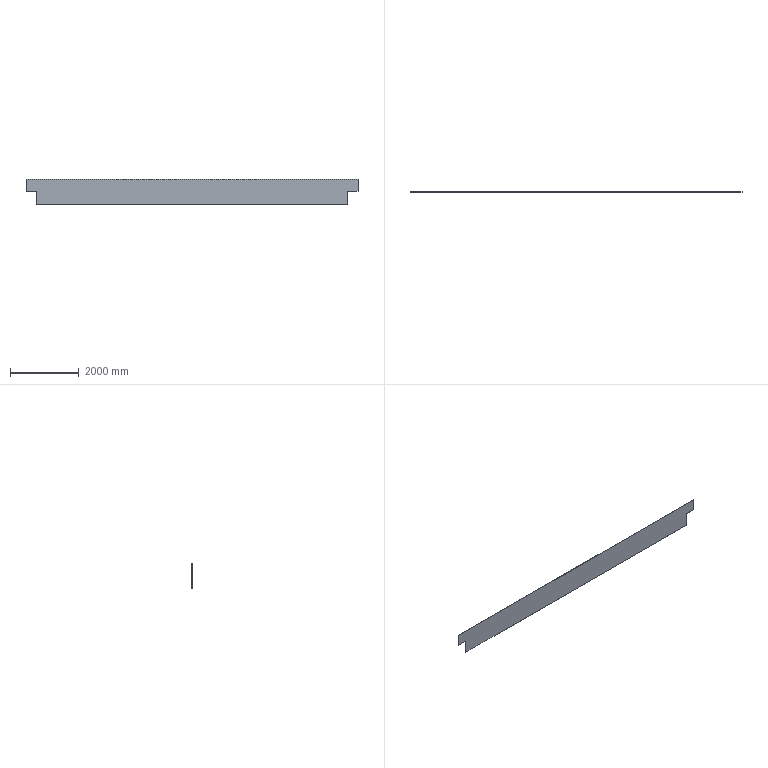Component | SolidWorks | Main-1_9940X9340X750X6-1 | 1 solid | 10 faces | box 9670 x 6 x 750 mm | volume 42075000 mm3 | plane 10 | material Plain Carbon Steel
STEP:
#1=COLOUR_RGB('',0.7922,0.8196,0.9333);
#2=FILL_AREA_STYLE_COLOUR('',#1);
#3=FILL_AREA_STYLE('',(#2));
#4=SURFACE_STYLE_FILL_AREA(#3);
#5=SURFACE_SIDE_STYLE('',(#4));
#6=SURFACE_STYLE_USAGE(.BOTH.,#5);
#7=PRESENTATION_STYLE_ASSIGNMENT((#6));
#8=CARTESIAN_POINT('',(-132.764,83.28,219.133));
#9=VERTEX_POINT('',#8);
#10=CARTESIAN_POINT('',(-132.764,83.28,205.353));
#11=VERTEX_POINT('',#10);
#12=CARTESIAN_POINT('',(-132.764,83.28,205.353));
#13=DIRECTION('',(0.,0.,-1.));
#14=VECTOR('',#13,39.37);
#15=LINE('',#12,#14);
#16=EDGE_CURVE('',#9,#11,#15,.T.);
#17=ORIENTED_EDGE('',*,*,#16,.F.);
#18=CARTESIAN_POINT('',(-132.764,83.517,219.133));
#19=VERTEX_POINT('',#18);
#20=CARTESIAN_POINT('',(-132.764,83.517,219.133));
#21=DIRECTION('',(0.,-1.,-0.));
#22=VECTOR('',#21,39.37);
#23=LINE('',#20,#22);
#24=EDGE_CURVE('',#19,#9,#23,.T.);
#25=ORIENTED_EDGE('',*,*,#24,.F.);
#26=CARTESIAN_POINT('',(-132.764,83.517,205.353));
#27=VERTEX_POINT('',#26);
#28=CARTESIAN_POINT('',(-132.764,83.517,205.353));
#29=DIRECTION('',(0.,0.,-1.));
#30=VECTOR('',#29,39.37);
#31=LINE('',#28,#30);
#32=EDGE_CURVE('',#19,#27,#31,.T.);
#33=ORIENTED_EDGE('',*,*,#32,.T.);
#34=CARTESIAN_POINT('',(-132.764,83.517,205.353));
#35=DIRECTION('',(0.,-1.,-0.));
#36=VECTOR('',#35,39.37);
#37=LINE('',#34,#36);
#38=EDGE_CURVE('',#27,#11,#37,.T.);
#39=ORIENTED_EDGE('',*,*,#38,.T.);
#40=EDGE_LOOP('',(#17,#25,#33,#39));
#41=FACE_OUTER_BOUND('',#40,.T.);
#42=CARTESIAN_POINT('',(-132.764,83.517,205.353));
#43=DIRECTION('',(-1.,0.,0.));
#44=DIRECTION('',(0.,0.,-1.));
#45=AXIS2_PLACEMENT_3D('',#42,#43,#44);
#46=PLANE('',#45);
#47=ADVANCED_FACE('',(#41),#46,.T.);
#48=CARTESIAN_POINT('',(247.945,83.28,219.133));
#49=VERTEX_POINT('',#48);
#50=CARTESIAN_POINT('',(-132.764,83.28,219.133));
#51=DIRECTION('',(-1.,0.,0.));
#52=VECTOR('',#51,39.37);
#53=LINE('',#50,#52);
#54=EDGE_CURVE('',#49,#9,#53,.T.);
#55=ORIENTED_EDGE('',*,*,#54,.F.);
#56=CARTESIAN_POINT('',(247.945,83.517,219.133));
#57=VERTEX_POINT('',#56);
#58=CARTESIAN_POINT('',(247.945,83.517,219.133));
#59=DIRECTION('',(0.,-1.,-0.));
#60=VECTOR('',#59,39.37);
#61=LINE('',#58,#60);
#62=EDGE_CURVE('',#57,#49,#61,.T.);
#63=ORIENTED_EDGE('',*,*,#62,.F.);
#64=CARTESIAN_POINT('',(-132.764,83.517,219.133));
#65=DIRECTION('',(-1.,0.,0.));
#66=VECTOR('',#65,39.37);
#67=LINE('',#64,#66);
#68=EDGE_CURVE('',#57,#19,#67,.T.);
#69=ORIENTED_EDGE('',*,*,#68,.T.);
#70=ORIENTED_EDGE('',*,*,#24,.T.);
#71=EDGE_LOOP('',(#55,#63,#69,#70));
#72=FACE_OUTER_BOUND('',#71,.T.);
#73=CARTESIAN_POINT('',(-132.764,83.517,219.133));
#74=DIRECTION('',(0.,-0.,1.));
#75=DIRECTION('',(-1.,0.,0.));
#76=AXIS2_PLACEMENT_3D('',#73,#74,#75);
#77=PLANE('',#76);
#78=ADVANCED_FACE('',(#72),#77,.T.);
#79=CARTESIAN_POINT('',(247.945,83.28,205.353));
#80=VERTEX_POINT('',#79);
#81=CARTESIAN_POINT('',(247.945,83.28,219.133));
#82=DIRECTION('',(0.,-0.,1.));
#83=VECTOR('',#82,39.37);
#84=LINE('',#81,#83);
#85=EDGE_CURVE('',#80,#49,#84,.T.);
#86=ORIENTED_EDGE('',*,*,#85,.F.);
#87=CARTESIAN_POINT('',(247.945,83.517,205.353));
#88=VERTEX_POINT('',#87);
#89=CARTESIAN_POINT('',(247.945,83.517,205.353));
#90=DIRECTION('',(0.,-1.,-0.));
#91=VECTOR('',#90,39.37);
#92=LINE('',#89,#91);
#93=EDGE_CURVE('',#88,#80,#92,.T.);
#94=ORIENTED_EDGE('',*,*,#93,.F.);
#95=CARTESIAN_POINT('',(247.945,83.517,219.133));
#96=DIRECTION('',(0.,-0.,1.));
#97=VECTOR('',#96,39.37);
#98=LINE('',#95,#97);
#99=EDGE_CURVE('',#88,#57,#98,.T.);
#100=ORIENTED_EDGE('',*,*,#99,.T.);
#101=ORIENTED_EDGE('',*,*,#62,.T.);
#102=EDGE_LOOP('',(#86,#94,#100,#101));
#103=FACE_OUTER_BOUND('',#102,.T.);
#104=CARTESIAN_POINT('',(247.945,83.517,219.133));
#105=DIRECTION('',(1.,0.,0.));
#106=DIRECTION('',(0.,-0.,1.));
#107=AXIS2_PLACEMENT_3D('',#104,#105,#106);
#108=PLANE('',#107);
#109=ADVANCED_FACE('',(#103),#108,.T.);
#110=CARTESIAN_POINT('',(236.134,83.28,205.353));
#111=VERTEX_POINT('',#110);
#112=CARTESIAN_POINT('',(247.945,83.28,205.353));
#113=DIRECTION('',(1.,0.,0.));
#114=VECTOR('',#113,39.37);
#115=LINE('',#112,#114);
#116=EDGE_CURVE('',#111,#80,#115,.T.);
#117=ORIENTED_EDGE('',*,*,#116,.F.);
#118=CARTESIAN_POINT('',(236.134,83.517,205.353));
#119=VERTEX_POINT('',#118);
#120=CARTESIAN_POINT('',(236.134,83.517,205.353));
#121=DIRECTION('',(0.,-1.,-0.));
#122=VECTOR('',#121,39.37);
#123=LINE('',#120,#122);
#124=EDGE_CURVE('',#119,#111,#123,.T.);
#125=ORIENTED_EDGE('',*,*,#124,.F.);
#126=CARTESIAN_POINT('',(247.945,83.517,205.353));
#127=DIRECTION('',(1.,0.,0.));
#128=VECTOR('',#127,39.37);
#129=LINE('',#126,#128);
#130=EDGE_CURVE('',#119,#88,#129,.T.);
#131=ORIENTED_EDGE('',*,*,#130,.T.);
#132=ORIENTED_EDGE('',*,*,#93,.T.);
#133=EDGE_LOOP('',(#117,#125,#131,#132));
#134=FACE_OUTER_BOUND('',#133,.T.);
#135=CARTESIAN_POINT('',(247.945,83.517,205.353));
#136=DIRECTION('',(0.,0.,-1.));
#137=DIRECTION('',(1.,0.,0.));
#138=AXIS2_PLACEMENT_3D('',#135,#136,#137);
#139=PLANE('',#138);
#140=ADVANCED_FACE('',(#134),#139,.T.);
#141=CARTESIAN_POINT('',(236.134,83.28,189.605));
#142=VERTEX_POINT('',#141);
#143=CARTESIAN_POINT('',(236.134,83.28,205.353));
#144=DIRECTION('',(0.,-0.,1.));
#145=VECTOR('',#144,39.37);
#146=LINE('',#143,#145);
#147=EDGE_CURVE('',#142,#111,#146,.T.);
#148=ORIENTED_EDGE('',*,*,#147,.F.);
#149=CARTESIAN_POINT('',(236.134,83.517,189.605));
#150=VERTEX_POINT('',#149);
#151=CARTESIAN_POINT('',(236.134,83.517,189.605));
#152=DIRECTION('',(0.,-1.,-0.));
#153=VECTOR('',#152,39.37);
#154=LINE('',#151,#153);
#155=EDGE_CURVE('',#150,#142,#154,.T.);
#156=ORIENTED_EDGE('',*,*,#155,.F.);
#157=CARTESIAN_POINT('',(236.134,83.517,205.353));
#158=DIRECTION('',(0.,-0.,1.));
#159=VECTOR('',#158,39.37);
#160=LINE('',#157,#159);
#161=EDGE_CURVE('',#150,#119,#160,.T.);
#162=ORIENTED_EDGE('',*,*,#161,.T.);
#163=ORIENTED_EDGE('',*,*,#124,.T.);
#164=EDGE_LOOP('',(#148,#156,#162,#163));
#165=FACE_OUTER_BOUND('',#164,.T.);
#166=CARTESIAN_POINT('',(236.134,83.517,205.353));
#167=DIRECTION('',(1.,0.,0.));
#168=DIRECTION('',(0.,-0.,1.));
#169=AXIS2_PLACEMENT_3D('',#166,#167,#168);
#170=PLANE('',#169);
#171=ADVANCED_FACE('',(#165),#170,.T.);
#172=CARTESIAN_POINT('',(-120.953,83.28,189.605));
#173=VERTEX_POINT('',#172);
#174=CARTESIAN_POINT('',(236.134,83.28,189.605));
#175=DIRECTION('',(1.,-0.,0.));
#176=VECTOR('',#175,39.37);
#177=LINE('',#174,#176);
#178=EDGE_CURVE('',#173,#142,#177,.T.);
#179=ORIENTED_EDGE('',*,*,#178,.F.);
#180=CARTESIAN_POINT('',(-120.953,83.517,189.605));
#181=VERTEX_POINT('',#180);
#182=CARTESIAN_POINT('',(-120.953,83.517,189.605));
#183=DIRECTION('',(0.,-1.,-0.));
#184=VECTOR('',#183,39.37);
#185=LINE('',#182,#184);
#186=EDGE_CURVE('',#181,#173,#185,.T.);
#187=ORIENTED_EDGE('',*,*,#186,.F.);
#188=CARTESIAN_POINT('',(236.134,83.517,189.605));
#189=DIRECTION('',(1.,-0.,0.));
#190=VECTOR('',#189,39.37);
#191=LINE('',#188,#190);
#192=EDGE_CURVE('',#181,#150,#191,.T.);
#193=ORIENTED_EDGE('',*,*,#192,.T.);
#194=ORIENTED_EDGE('',*,*,#155,.T.);
#195=EDGE_LOOP('',(#179,#187,#193,#194));
#196=FACE_OUTER_BOUND('',#195,.T.);
#197=CARTESIAN_POINT('',(236.134,83.517,189.605));
#198=DIRECTION('',(0.,0.,-1.));
#199=DIRECTION('',(1.,-0.,0.));
#200=AXIS2_PLACEMENT_3D('',#197,#198,#199);
#201=PLANE('',#200);
#202=ADVANCED_FACE('',(#196),#201,.T.);
#203=CARTESIAN_POINT('',(-120.953,83.28,205.353));
#204=VERTEX_POINT('',#203);
#205=CARTESIAN_POINT('',(-120.953,83.28,189.605));
#206=DIRECTION('',(0.,0.,-1.));
#207=VECTOR('',#206,39.37);
#208=LINE('',#205,#207);
#209=EDGE_CURVE('',#204,#173,#208,.T.);
#210=ORIENTED_EDGE('',*,*,#209,.F.);
#211=CARTESIAN_POINT('',(-120.953,83.517,205.353));
#212=VERTEX_POINT('',#211);
#213=CARTESIAN_POINT('',(-120.953,83.517,205.353));
#214=DIRECTION('',(0.,-1.,-0.));
#215=VECTOR('',#214,39.37);
#216=LINE('',#213,#215);
#217=EDGE_CURVE('',#212,#204,#216,.T.);
#218=ORIENTED_EDGE('',*,*,#217,.F.);
#219=CARTESIAN_POINT('',(-120.953,83.517,189.605));
#220=DIRECTION('',(0.,0.,-1.));
#221=VECTOR('',#220,39.37);
#222=LINE('',#219,#221);
#223=EDGE_CURVE('',#212,#181,#222,.T.);
#224=ORIENTED_EDGE('',*,*,#223,.T.);
#225=ORIENTED_EDGE('',*,*,#186,.T.);
#226=EDGE_LOOP('',(#210,#218,#224,#225));
#227=FACE_OUTER_BOUND('',#226,.T.);
#228=CARTESIAN_POINT('',(-120.953,83.517,189.605));
#229=DIRECTION('',(-1.,0.,0.));
#230=DIRECTION('',(0.,0.,-1.));
#231=AXIS2_PLACEMENT_3D('',#228,#229,#230);
#232=PLANE('',#231);
#233=ADVANCED_FACE('',(#227),#232,.T.);
#234=CARTESIAN_POINT('',(-120.953,83.28,205.353));
#235=DIRECTION('',(1.,0.,0.));
#236=VECTOR('',#235,39.37);
#237=LINE('',#234,#236);
#238=EDGE_CURVE('',#11,#204,#237,.T.);
#239=ORIENTED_EDGE('',*,*,#238,.F.);
#240=ORIENTED_EDGE('',*,*,#38,.F.);
#241=CARTESIAN_POINT('',(-120.953,83.517,205.353));
#242=DIRECTION('',(1.,0.,0.));
#243=VECTOR('',#242,39.37);
#244=LINE('',#241,#243);
#245=EDGE_CURVE('',#27,#212,#244,.T.);
#246=ORIENTED_EDGE('',*,*,#245,.T.);
#247=ORIENTED_EDGE('',*,*,#217,.T.);
#248=EDGE_LOOP('',(#239,#240,#246,#247));
#249=FACE_OUTER_BOUND('',#248,.T.);
#250=CARTESIAN_POINT('',(-120.953,83.517,205.353));
#251=DIRECTION('',(0.,0.,-1.));
#252=DIRECTION('',(1.,0.,0.));
#253=AXIS2_PLACEMENT_3D('',#250,#251,#252);
#254=PLANE('',#253);
#255=ADVANCED_FACE('',(#249),#254,.T.);
#256=ORIENTED_EDGE('',*,*,#32,.F.);
#257=ORIENTED_EDGE('',*,*,#68,.F.);
#258=ORIENTED_EDGE('',*,*,#99,.F.);
#259=ORIENTED_EDGE('',*,*,#130,.F.);
#260=ORIENTED_EDGE('',*,*,#161,.F.);
#261=ORIENTED_EDGE('',*,*,#192,.F.);
#262=ORIENTED_EDGE('',*,*,#223,.F.);
#263=ORIENTED_EDGE('',*,*,#245,.F.);
#264=EDGE_LOOP('',(#256,#257,#258,#259,#260,#261,#262,#263));
#265=FACE_OUTER_BOUND('',#264,.T.);
#266=CARTESIAN_POINT('',(-132.764,83.517,219.133));
#267=DIRECTION('',(0.,1.,0.));
#268=DIRECTION('',(0.,-0.,1.));
#269=AXIS2_PLACEMENT_3D('',#266,#267,#268);
#270=PLANE('',#269);
#271=ADVANCED_FACE('',(#265),#270,.T.);
#272=ORIENTED_EDGE('',*,*,#16,.T.);
#273=ORIENTED_EDGE('',*,*,#238,.T.);
#274=ORIENTED_EDGE('',*,*,#209,.T.);
#275=ORIENTED_EDGE('',*,*,#178,.T.);
#276=ORIENTED_EDGE('',*,*,#147,.T.);
#277=ORIENTED_EDGE('',*,*,#116,.T.);
#278=ORIENTED_EDGE('',*,*,#85,.T.);
#279=ORIENTED_EDGE('',*,*,#54,.T.);
#280=EDGE_LOOP('',(#272,#273,#274,#275,#276,#277,#278,#279));
#281=FACE_OUTER_BOUND('',#280,.T.);
#282=CARTESIAN_POINT('',(-132.764,83.28,219.133));
#283=DIRECTION('',(0.,1.,0.));
#284=DIRECTION('',(0.,-0.,1.));
#285=AXIS2_PLACEMENT_3D('',#282,#283,#284);
#286=PLANE('',#285);
#287=ADVANCED_FACE('',(#281),#286,.F.);
#288=CLOSED_SHELL('',(#47,#78,#109,#140,#171,#202,#233,#255,#271,#287));
#289=MANIFOLD_SOLID_BREP('',#288);
#290=STYLED_ITEM('',(#7),#289);
#291=PRESENTATION_LAYER_ASSIGNMENT('','',(#290));
#292=CARTESIAN_POINT('',(0.,0.,0.));
#293=DIRECTION('',(0.,0.,1.));
#294=DIRECTION('',(1.,0.,0.));
#295=AXIS2_PLACEMENT_3D('',#292,#293,#294);
#296=(LENGTH_UNIT()NAMED_UNIT(*)SI_UNIT($,.METRE.));
#297=LENGTH_MEASURE_WITH_UNIT(LENGTH_MEASURE(0.0254),#296);
#298=DIMENSIONAL_EXPONENTS(1.,0.,0.,0.,0.,0.,0.);
#299=(CONVERSION_BASED_UNIT('',#297)LENGTH_UNIT()NAMED_UNIT(#298));
#300=UNCERTAINTY_MEASURE_WITH_UNIT(LENGTH_MEASURE(0.00001),#299,'','');
#301=(NAMED_UNIT(*)PLANE_ANGLE_UNIT()SI_UNIT($,.RADIAN.));
#302=(NAMED_UNIT(*)SI_UNIT($,.STERADIAN.)SOLID_ANGLE_UNIT());
#303=(GEOMETRIC_REPRESENTATION_CONTEXT(3)GLOBAL_UNCERTAINTY_ASSIGNED_CONTEXT((#300))GLOBAL_UNIT_ASSIGNED_CONTEXT((#299,#301,#302))REPRESENTATION_CONTEXT('',''));
#304=ADVANCED_BREP_SHAPE_REPRESENTATION('',(#289,#295),#303);
#305=(LENGTH_UNIT()NAMED_UNIT(*)SI_UNIT($,.METRE.));
#306=LENGTH_MEASURE_WITH_UNIT(LENGTH_MEASURE(0.0254),#305);
#307=DIMENSIONAL_EXPONENTS(1.,0.,0.,0.,0.,0.,0.);
#308=(CONVERSION_BASED_UNIT('',#306)LENGTH_UNIT()NAMED_UNIT(#307));
#309=UNCERTAINTY_MEASURE_WITH_UNIT(LENGTH_MEASURE(0.00001),#308,'','');
#310=(NAMED_UNIT(*)PLANE_ANGLE_UNIT()SI_UNIT($,.RADIAN.));
#311=(NAMED_UNIT(*)SI_UNIT($,.STERADIAN.)SOLID_ANGLE_UNIT());
#312=(GEOMETRIC_REPRESENTATION_CONTEXT(3)GLOBAL_UNCERTAINTY_ASSIGNED_CONTEXT((#309))GLOBAL_UNIT_ASSIGNED_CONTEXT((#308,#310,#311))REPRESENTATION_CONTEXT('',''));
#313=MECHANICAL_DESIGN_GEOMETRIC_PRESENTATION_REPRESENTATION('',(#290),#312);